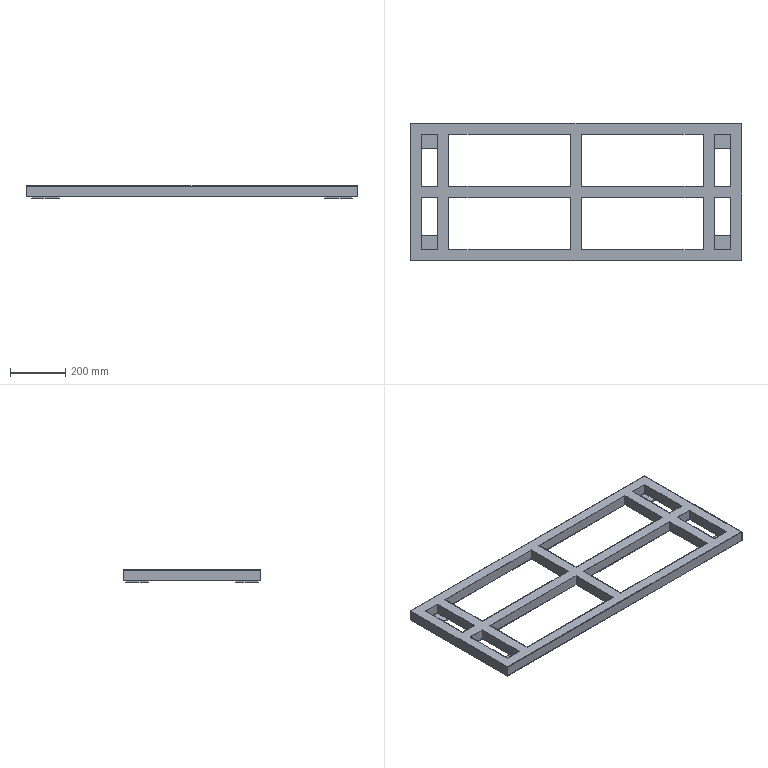Component | SolidWorks | CartChassis-1_ChassisFrame-1 | 1 solid | 104 faces | box 1197 x 497 x 46 mm | volume 1451293 mm3 | plane 104 | material Q235-A
build123d program:
from build123d import *

# Parameters (mm, degrees)
SKETCH1_W           = 1197
SKETCH1_H           = 497
SKETCH1_W_2         = 60
SKETCH1_H_2         = 188.5
SKETCH1_W_3         = 438.5
BOSS_EXTRUDE1_DEPTH = 40
SHELL1_T            = -1.5
SKETCH2_W           = 40
SKETCH2_H           = 497
BOSS_EXTRUDE2_DEPTH = 3
SKETCH3_W           = 100
SKETCH3_H           = 80
BOSS_EXTRUDE3_DEPTH = 6
CHAMFER1_SIZE       = 1.6


with BuildPart() as part:
    # Sketch1 → Boss-Extrude1 (new body)
    with BuildSketch(Plane.XY):
        Rectangle(SKETCH1_W, SKETCH1_H)
        with Locations((-528.5, 114.25)):
            Rectangle(SKETCH1_W_2, SKETCH1_H_2, mode=Mode.SUBTRACT)
        with Locations((528.5, -114.25)):
            Rectangle(SKETCH1_W_2, SKETCH1_H_2, mode=Mode.SUBTRACT)
        with Locations((-528.5, -114.25)):
            Rectangle(SKETCH1_W_2, SKETCH1_H_2, mode=Mode.SUBTRACT)
        with Locations((-239.25, 114.25)):
            Rectangle(SKETCH1_W_3, SKETCH1_H_2, mode=Mode.SUBTRACT)
        with Locations((-239.25, -114.25)):
            Rectangle(SKETCH1_W_3, SKETCH1_H_2, mode=Mode.SUBTRACT)
        with Locations((528.5, 114.25)):
            Rectangle(SKETCH1_W_2, SKETCH1_H_2, mode=Mode.SUBTRACT)
        with Locations((239.25, 114.25)):
            Rectangle(SKETCH1_W_3, SKETCH1_H_2, mode=Mode.SUBTRACT)
        with Locations((239.25, -114.25)):
            Rectangle(SKETCH1_W_3, SKETCH1_H_2, mode=Mode.SUBTRACT)
    extrude(amount=BOSS_EXTRUDE1_DEPTH)

    # Shell1
    shell1_openings = [part.faces().sort_by_distance(p)[0] for p in [
        (598.5, 0, 20),
    ]]
    offset(amount=SHELL1_T, openings=shell1_openings, kind=Kind.INTERSECTION)

    # Sketch2 → Boss-Extrude2 (add)
    with BuildSketch(Plane(origin=(598.5, 0, 0), x_dir=(0, 0, -1), z_dir=(1, 0, 0))):
        with Locations((-20, 0)):
            Rectangle(SKETCH2_W, SKETCH2_H)
    extrude(amount=-BOSS_EXTRUDE2_DEPTH)

    # Sketch3 → Boss-Extrude3 (add)
    with BuildSketch(Plane(origin=(0, 0, 0), x_dir=(-1, 0, 0), z_dir=(0, 0, -1))):
        with Locations((-528.5, 198.5)):
            Rectangle(SKETCH3_W, SKETCH3_H)
        with Locations((-528.5, -198.5)):
            Rectangle(SKETCH3_W, SKETCH3_H)
        with Locations((528.5, -198.5)):
            Rectangle(SKETCH3_W, SKETCH3_H)
        with Locations((528.5, 198.5)):
            Rectangle(SKETCH3_W, SKETCH3_H)
    extrude(amount=BOSS_EXTRUDE3_DEPTH)

    # Chamfer1
    chamfer1_edges = [part.edges().sort_by_distance(p)[0] for p in [
        (-598.5, 0, 40),
        (0, -248.5, 40),
        (598.5, 0, 40),
        (0, 248.5, 40),
    ]]
    chamfer(chamfer1_edges, length=CHAMFER1_SIZE)


solid = part.part

# Placed as in the assembly
solid = solid.moved(Location((-59.368, 33.925, 1182.25), (0, 0, 0)))